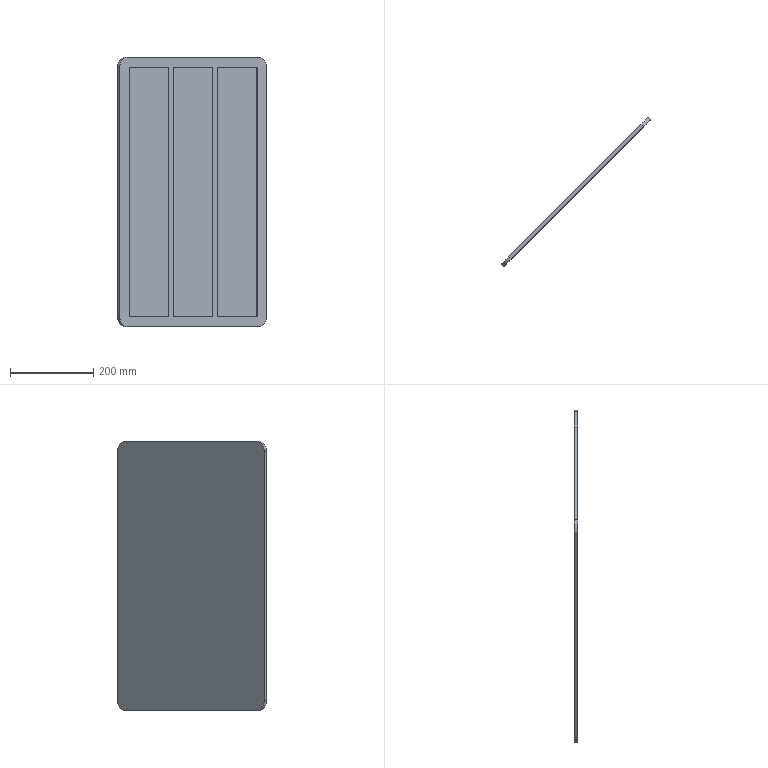Component | NX | PEDAL_2 | 1 solid | 25 faces | volume 2109708 mm3 | plane 21 | cylinder 4 | commonest cylinder face diameters 50 x4